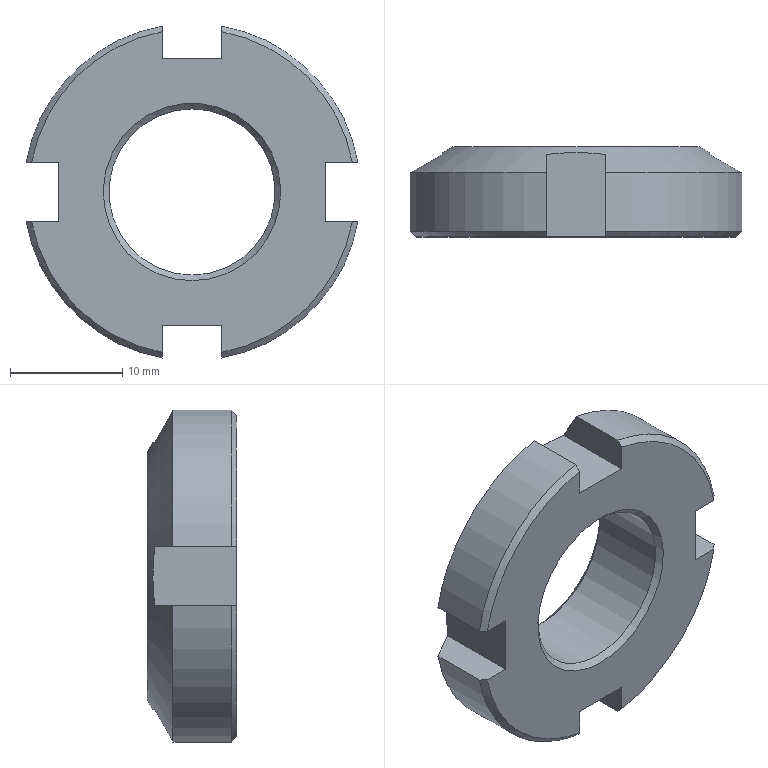Component | NX | GB812-88_M16X1_5 | 1 solid | 26 faces | volume 3444 mm3 | plane 14 | cone 7 | cylinder 5 | commonest cylinder face diameters 30 x4 14.782 x1